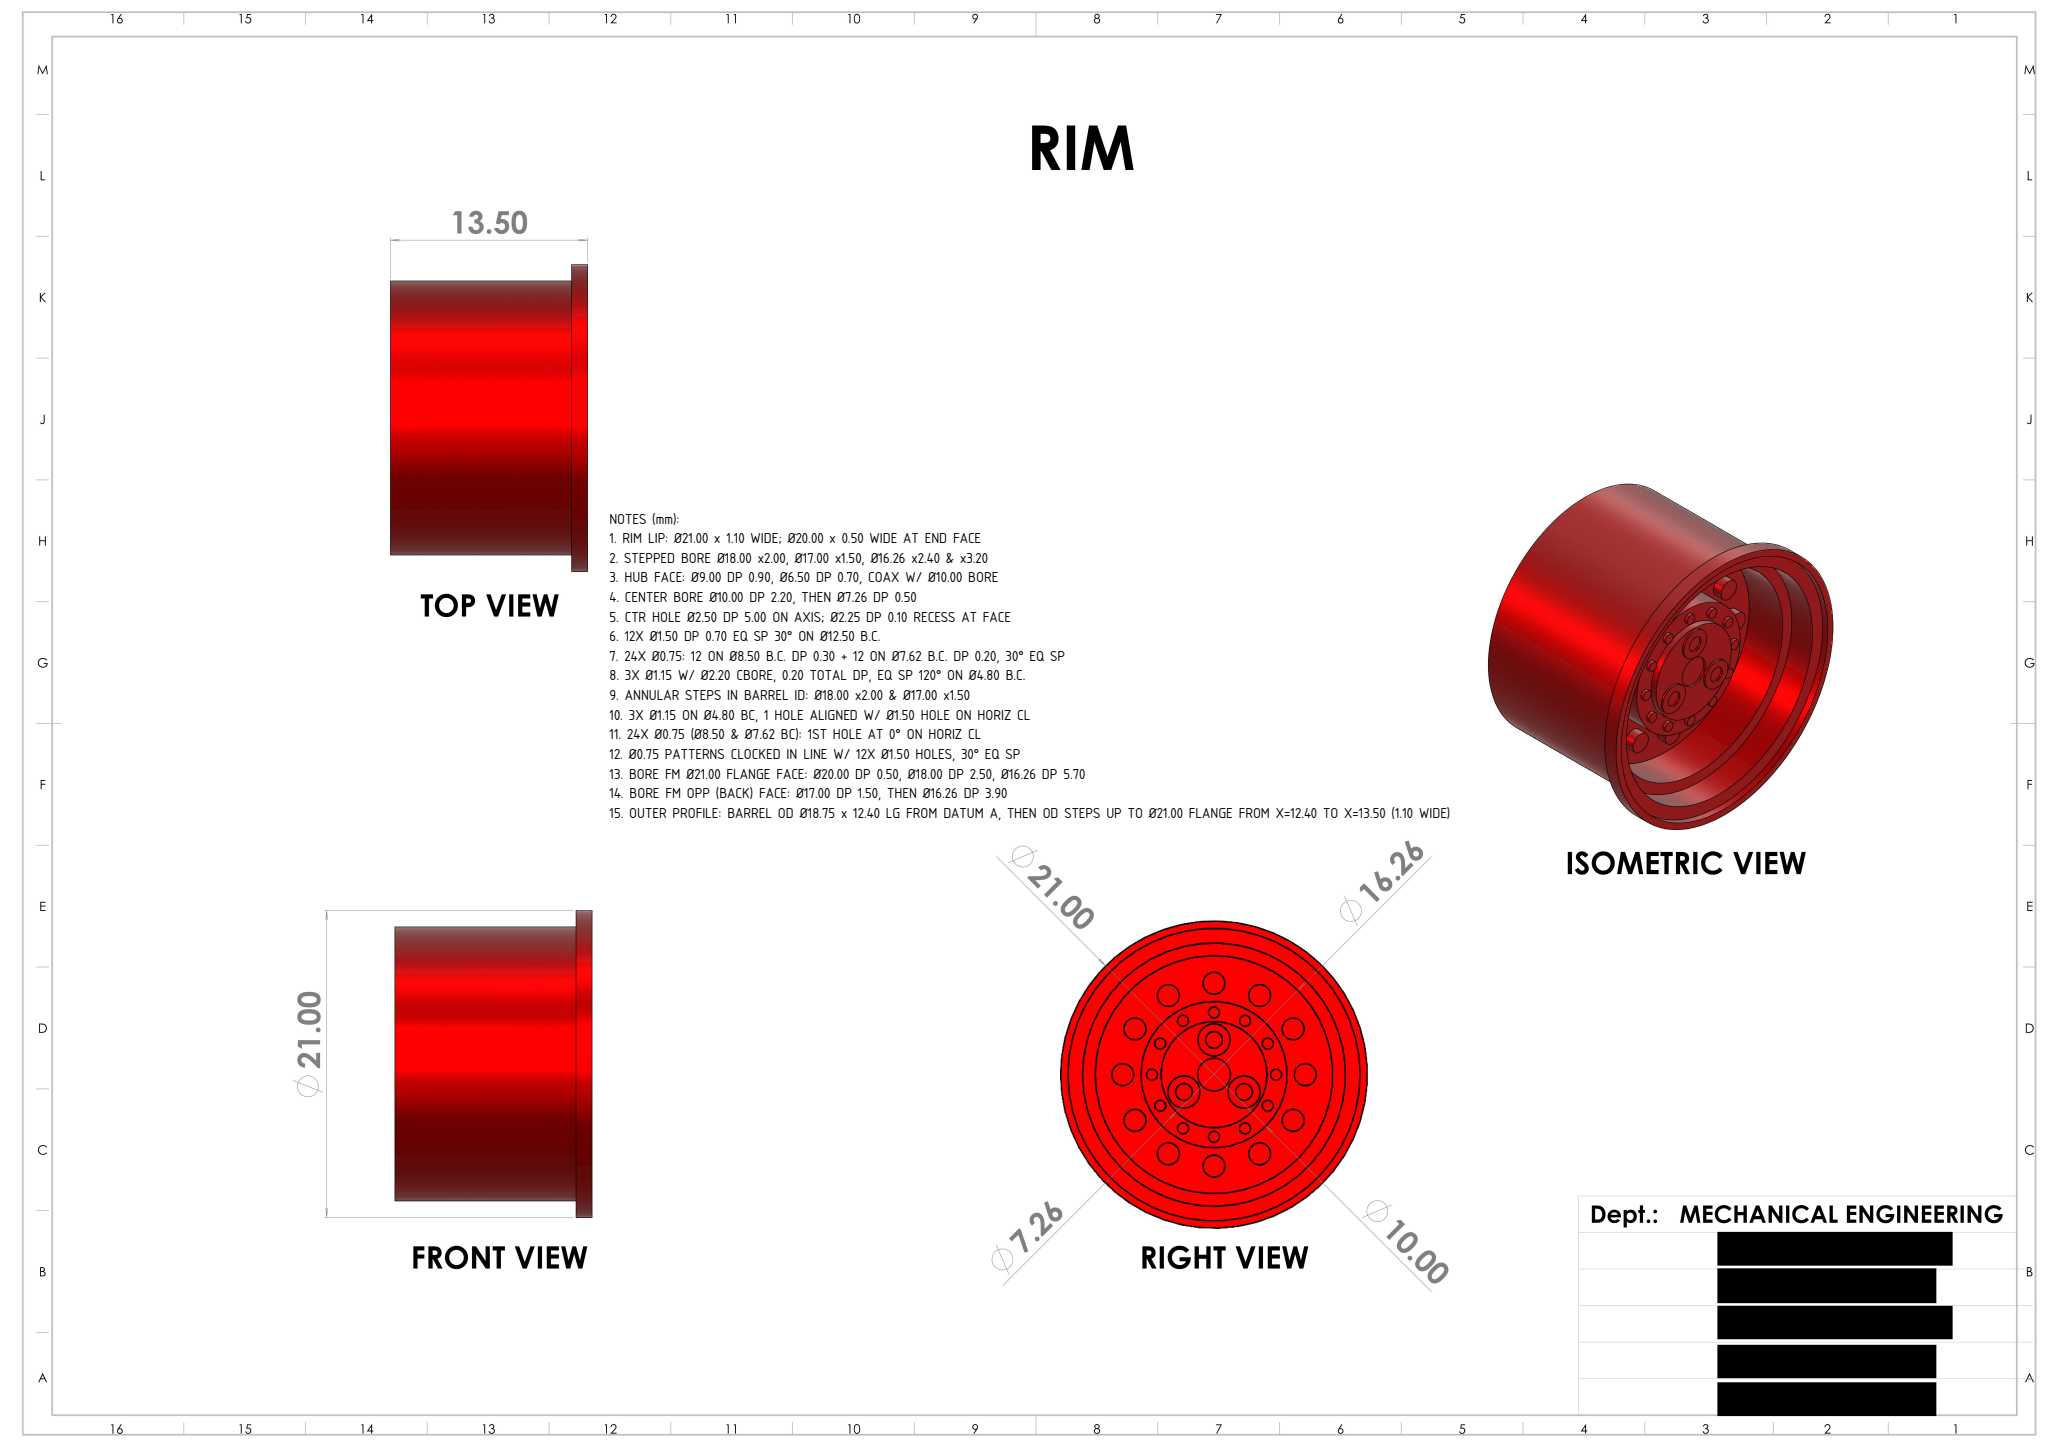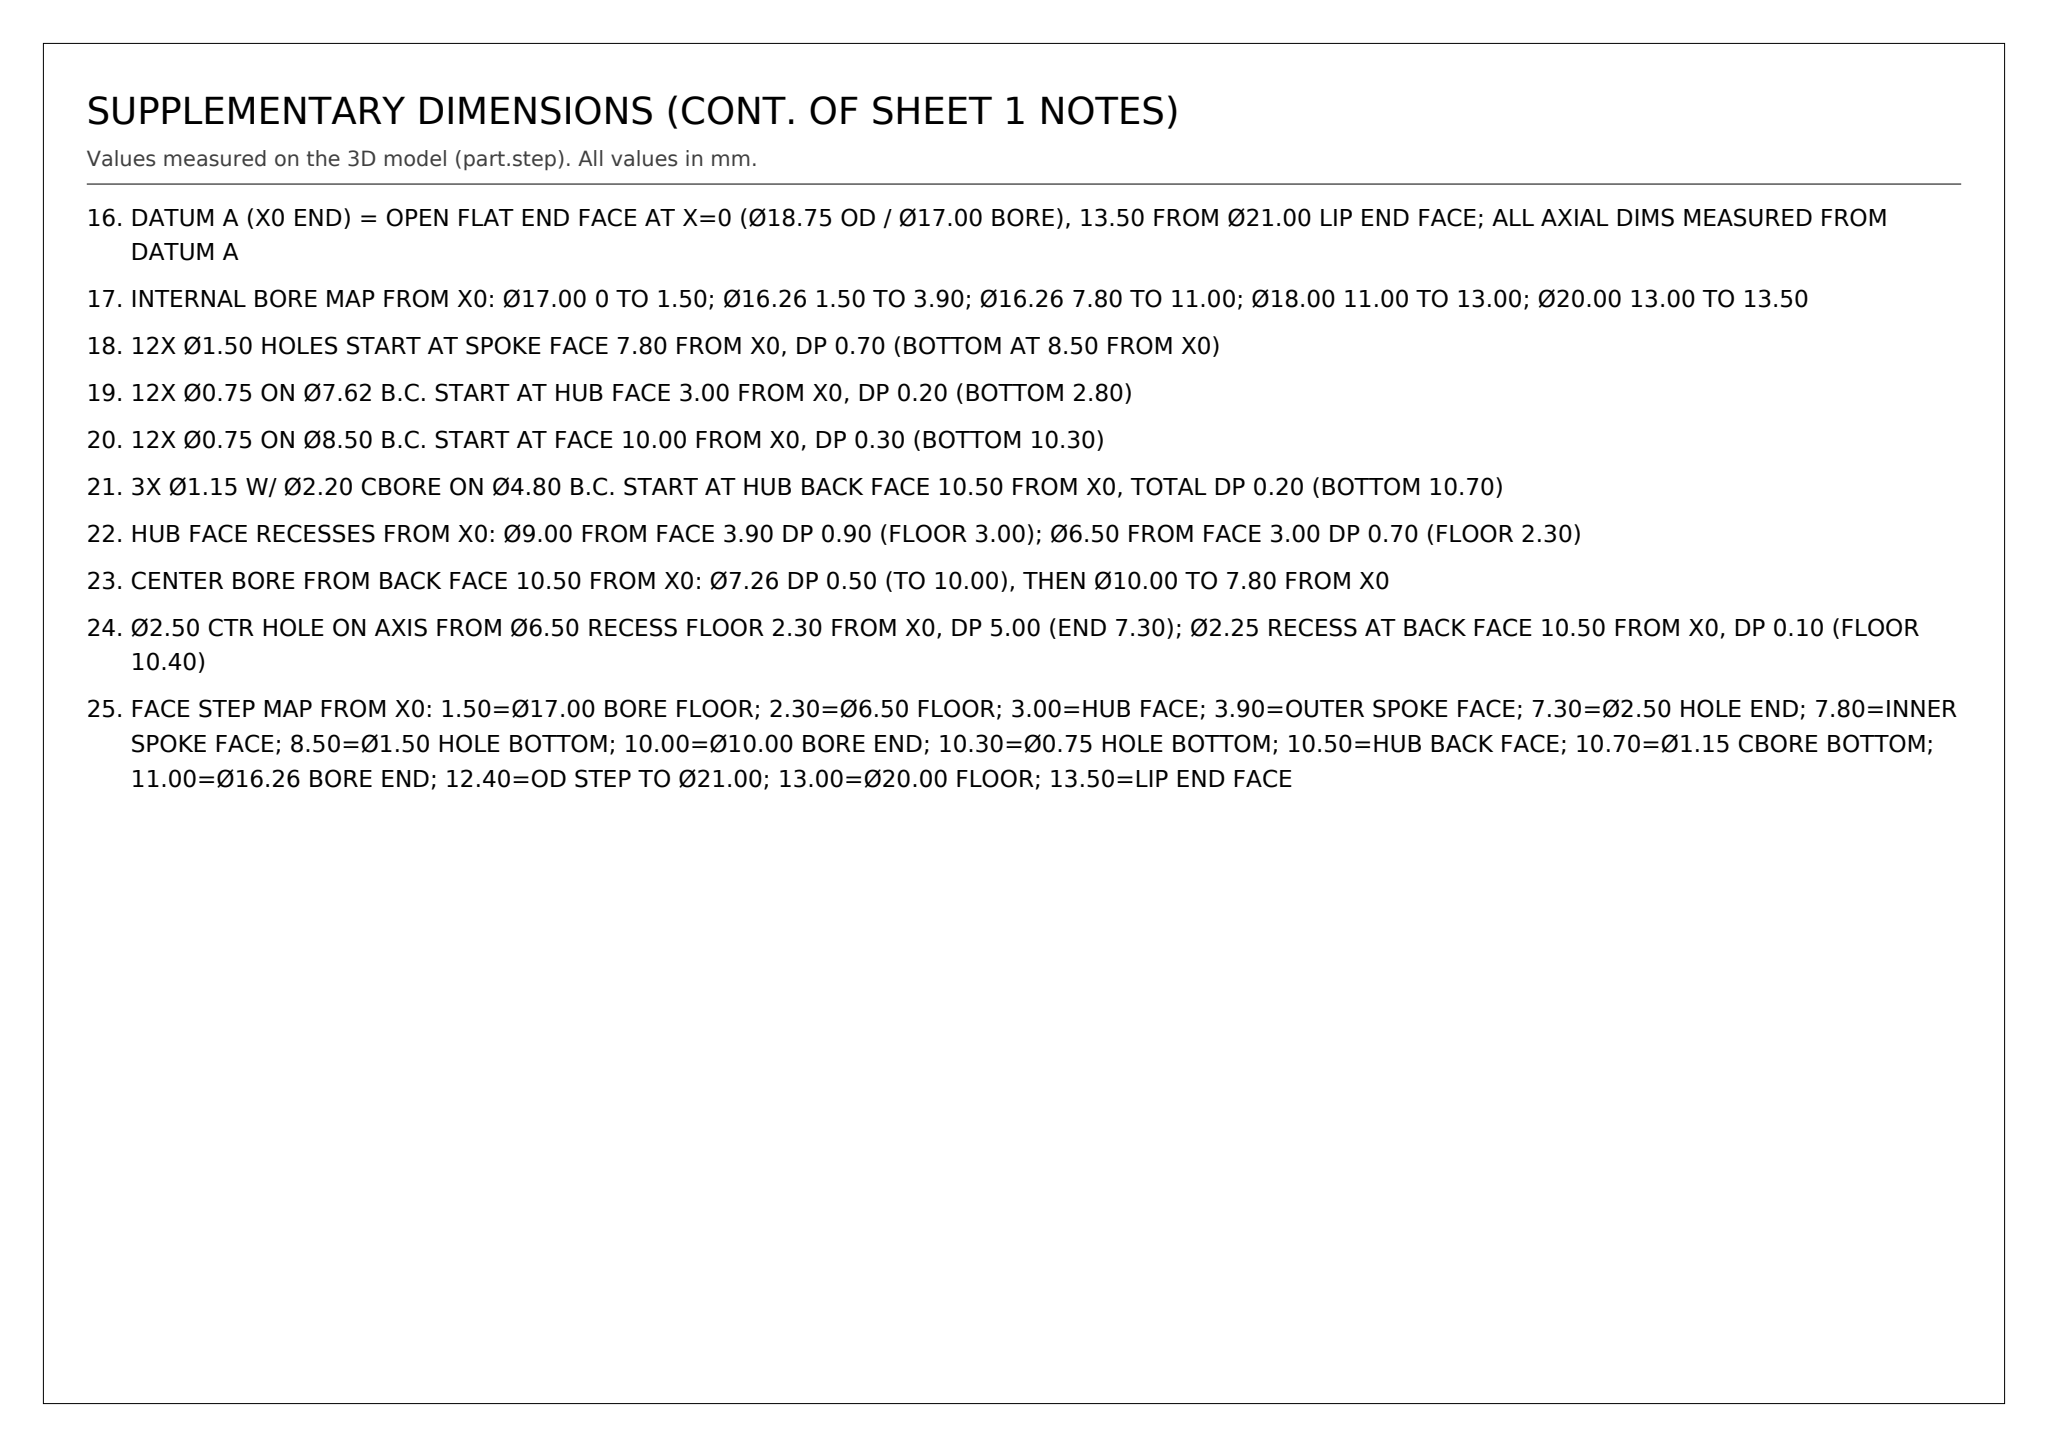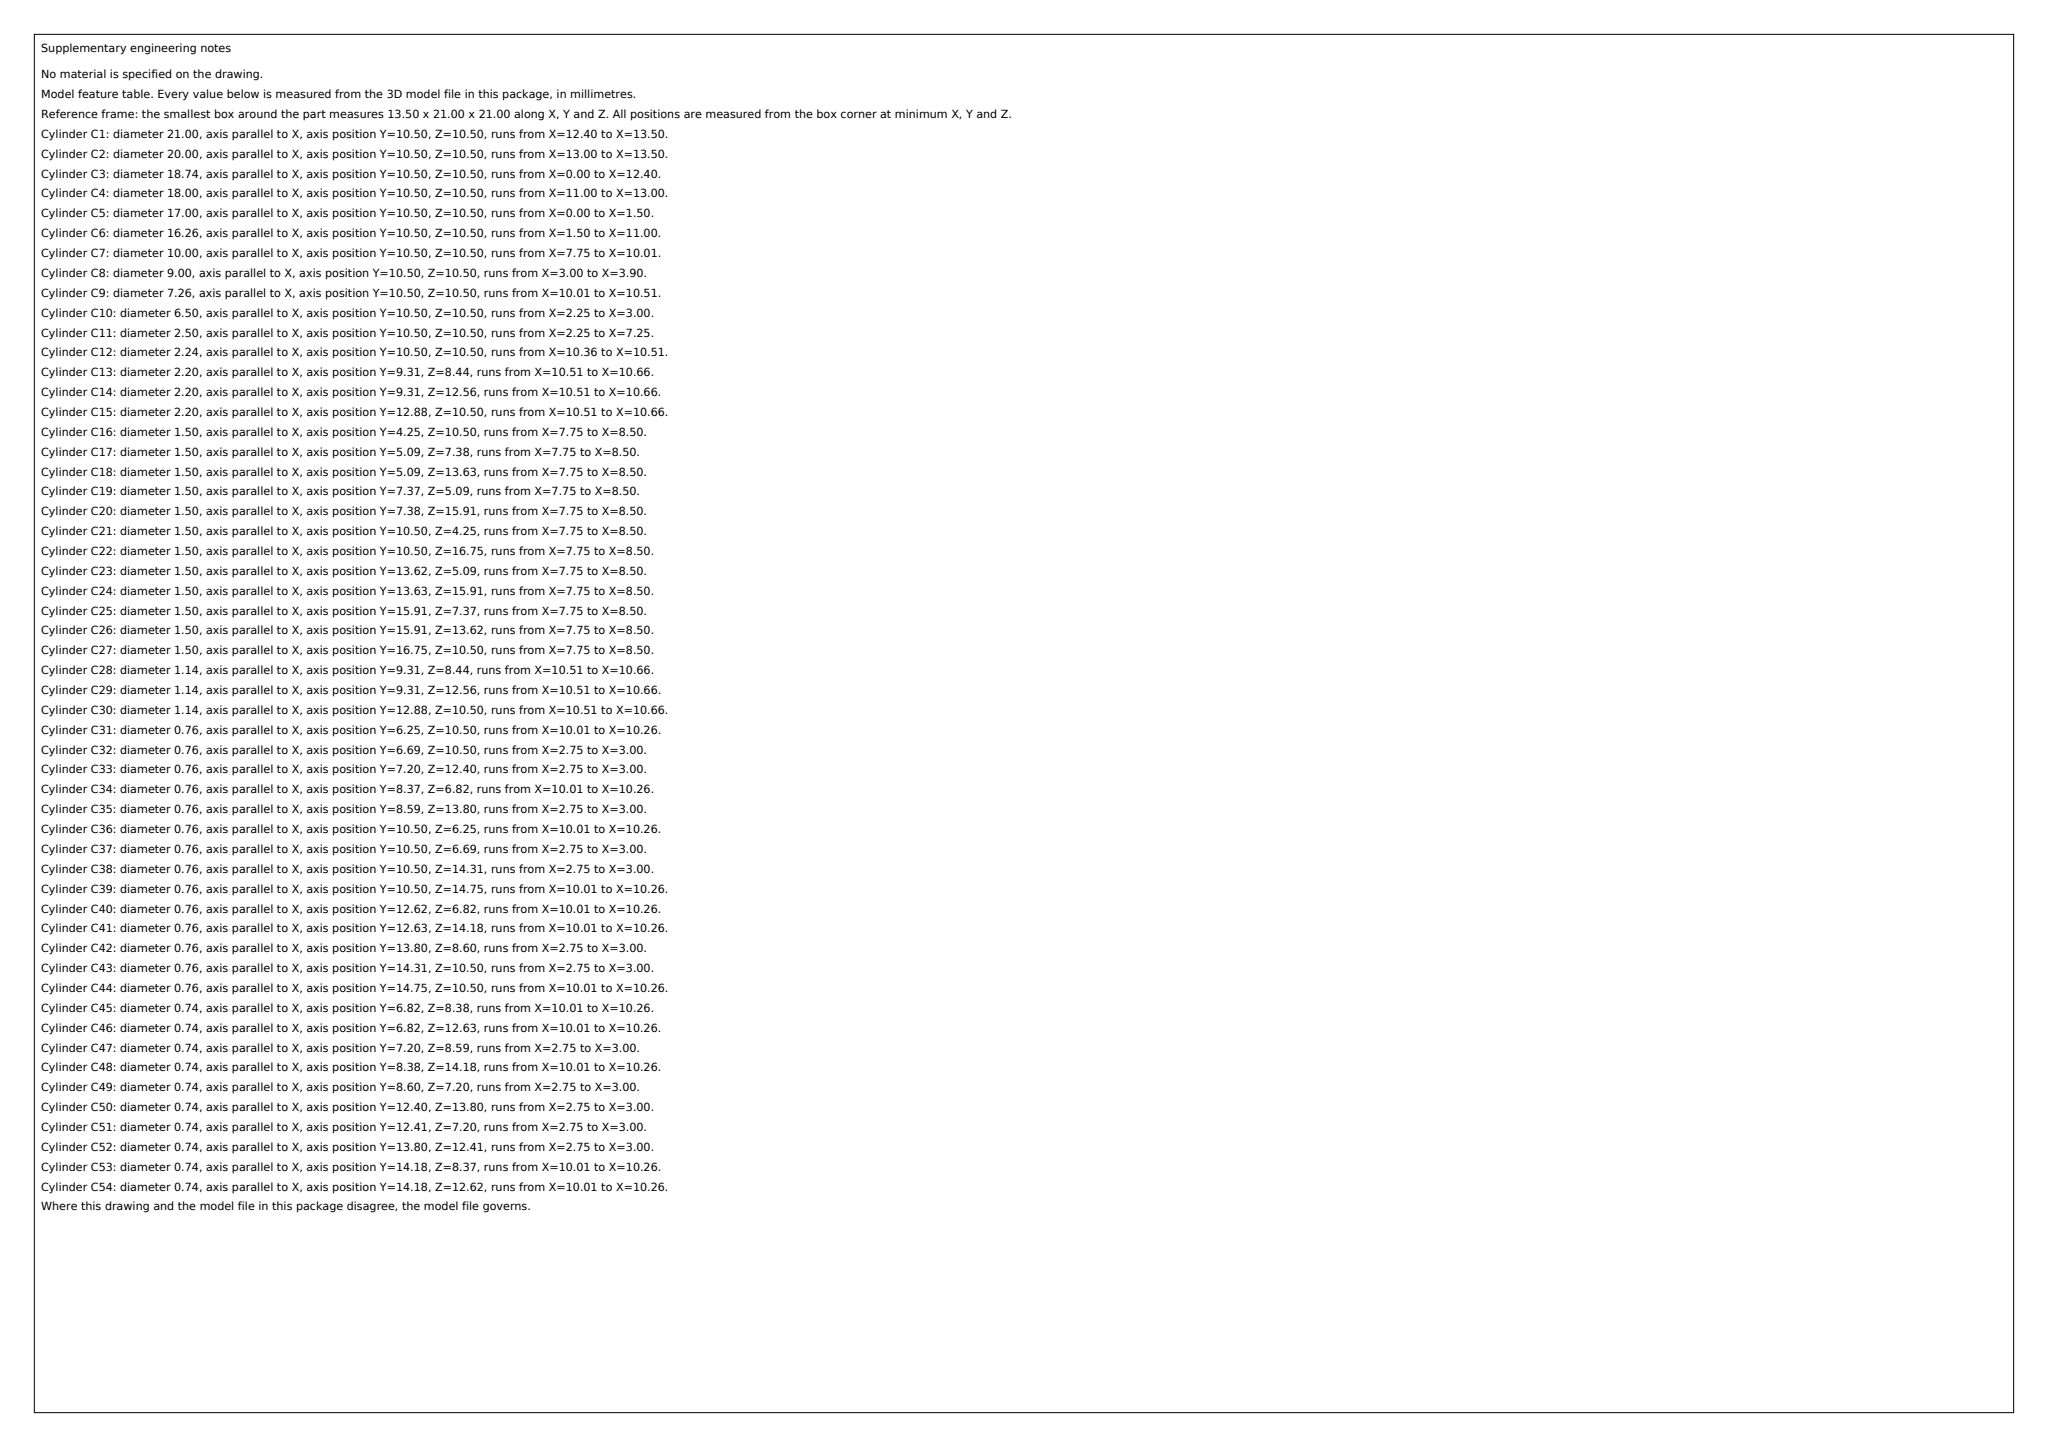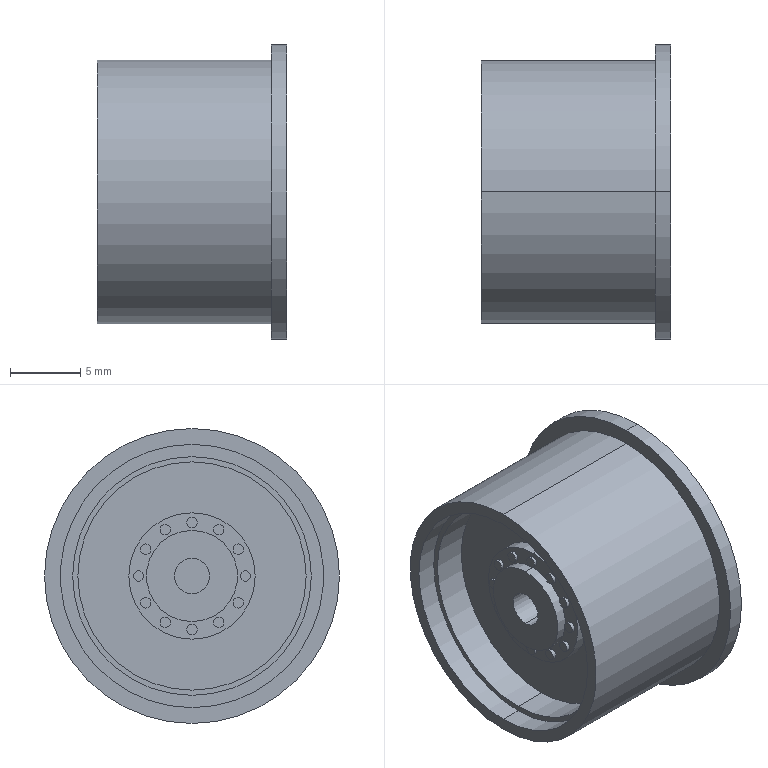Part | SolidWorks | mm | 1 solid | 166 faces | box 13.5 x 21 x 21 mm | volume 1900 mm3 | cylinder 110 | plane 56 | commonest cylinder face diameters 0.75 x48 1.5 x24 1.15 x6 2.2 x6 16.26 x4 2.5 x2 2.25 x2 21 x2
Drawing notes:
RIM LIP: Ø21.00 x 1.10 WIDE; Ø20.00 x 0.50 WIDE AT END FACE | from the solid: cyl [21.0,len 1.10] & [20.0,len 0.50]; planes x=12.40, 13.00, 13.50
STEPPED BORE Ø18.00 x2.00, Ø17.00 x1.50, Ø16.26 x2.40 & x3.20 | from the solid: bores: Ø18.00 x 11.00-13.00 (2.00); Ø17.00 x 0-1.50 (1.50); Ø16.26 x 1.50-3.90 (2.40) and x 7.80-11.00 (3.20)
HUB FACE: Ø9.00 DP 0.90, Ø6.50 DP 0.70, COAX W/ Ø10.00 BORE | from the solid: Ø9.00 x 3.00-3.90 (0.90); Ø6.50 x 2.30-3.00 (0.70); Ø10.00 bore x 7.80-10.00, all on axis y10.5 z10.5
CENTER BORE Ø10.00 DP 2.20, THEN Ø7.26 DP 0.50 | from the solid: Ø10.00 x 7.80-10.00 (2.20); Ø7.26 x 10.00-10.50 (0.50)
CTR HOLE Ø2.50 DP 5.00 ON AXIS; Ø2.25 DP 0.10 RECESS AT FACE | from the solid: Ø2.50 bore x 2.30-7.30 (5.00); Ø2.25 bore x 10.40-10.50 (0.10)
12X Ø1.50 DP 0.70 EQ SP 30° ON Ø12.50 B.C. | from the solid: 12X Ø1.50 x 7.80-8.50 (0.70), centers at radius 6.25 from axis (e.g. y10.5 z16.8; y15.9 z13.6)
24X Ø0.75: 12 ON Ø8.50 B.C. DP 0.30 + 12 ON Ø7.62 B.C. DP 0.20, 30° EQ SP | from the solid: 12X Ø0.75 x 10.00-10.30 (0.30) at r=4.25; 12X Ø0.75 x 2.80-3.00 (0.20) at r=3.81
3X Ø1.15 W/ Ø2.20 CBORE, 0.20 TOTAL DP, EQ SP 120° ON Ø4.80 B.C. | from the solid: 3X Ø2.20 and Ø1.15 x 10.50-10.70 (0.20) at (y12.9 z10.5), (y9.3 z12.6), (y9.3 z8.4) = r 2.40
ANNULAR STEPS IN BARREL ID: Ø18.00 x2.00 & Ø17.00 x1.50 | from the solid: cyls [18.0,len 2.0],[17.0,len 1.5] coax with Ø18.75 bore
3X Ø1.15 ON Ø4.80 BC, 1 HOLE ALIGNED W/ Ø1.50 HOLE ON HORIZ CL | from the solid: Ø1.15 holes at r=2.40 from axis (y12.9 z10.5 etc.), one at z=10.5 in line with Ø1.50 hole at y16.8 z10.5
24X Ø0.75 (Ø8.50 & Ø7.62 BC): 1ST HOLE AT 0° ON HORIZ CL | from the solid: Ø0.75 holes at r=4.25 (Ø8.50 BC) and r=3.81 (Ø7.62 BC) about center y10.5 z10.5; both sets at 0,30,60...330° (e.g. 14.75,10.5 and 14.31,10.5 on +Y horiz CL)
Ø0.75 PATTERNS CLOCKED IN LINE W/ 12X Ø1.50 HOLES, 30° EQ SP | from the solid: Ø1.50 holes r=6.25 at (16.75,10.5)=0°,(15.91,13.63)=30°...; same 0° start as both Ø0.75 bolt circles
BORE FM Ø21.00 FLANGE FACE: Ø20.00 DP 0.50, Ø18.00 DP 2.50, Ø16.26 DP 5.70 | from the solid: from x=13.50: Ø20.00 to 13.00 (0.50); Ø18.00 to 11.00 (2.50); Ø16.26 to 7.80 (5.70)
BORE FM OPP (BACK) FACE: Ø17.00 DP 1.50, THEN Ø16.26 DP 3.90 | from the solid: planes x0/1.5 = Ø17.00 x1.50; x1.5/3.9 = Ø16.26 x2.40; back face = x0, Ø18.75 barrel runs x0-12.4
OUTER PROFILE: BARREL OD Ø18.75 x 12.40 LG FROM DATUM A, THEN OD STEPS UP TO Ø21.00 FLANGE FROM X=12.40 TO X=13.50 (1.10 WIDE) | from the solid: cylinders Ø18.75 axis x L12.40 and Ø21.00 axis x L1.10; axis_plane x=12.4
DATUM A (X0 END) = OPEN FLAT END FACE AT X=0 (Ø18.75 OD / Ø17.00 BORE), 13.50 FROM Ø21.00 LIP END FACE; ALL AXIAL DIMS MEASURED FROM DATUM A | from the solid: axis_planes x=0.0 (extent y,z 1.1-19.9) and x=13.5; bbox_xyz x=13.50
INTERNAL BORE MAP FROM X0: Ø17.00 0 TO 1.50; Ø16.26 1.50 TO 3.90; Ø16.26 7.80 TO 11.00; Ø18.00 11.00 TO 13.00; Ø20.00 13.00 TO 13.50 | from the solid: hole/bore Ø17.0 x 0.0-1.5; Ø16.26 x 1.5-3.9; Ø16.26 x 7.8-11.0; Ø18.0 x 11.0-13.0; Ø20.0 x 13.0-13.5
12X Ø1.50 HOLES START AT SPOKE FACE 7.80 FROM X0, DP 0.70 (BOTTOM AT 8.50 FROM X0) | from the solid: cylinders Ø1.5 axis x from 7.8 to 8.5 (12 instances); axis_planes x=7.8 and x=8.5 pockets
12X Ø0.75 ON Ø7.62 B.C. START AT HUB FACE 3.00 FROM X0, DP 0.20 (BOTTOM 2.80) | from the solid: cylinders Ø0.75 axis x from 2.8 to 3.0 (12 instances, radius 3.8 from axis y10.5 z10.5); axis_plane x=3.0
12X Ø0.75 ON Ø8.50 B.C. START AT FACE 10.00 FROM X0, DP 0.30 (BOTTOM 10.30) | from the solid: cylinders Ø0.75 axis x from 10.0 to 10.3 (12 instances, radius ~4.3 from axis y10.5 z10.5); axis_plane x=10.0
3X Ø1.15 W/ Ø2.20 CBORE ON Ø4.80 B.C. START AT HUB BACK FACE 10.50 FROM X0, TOTAL DP 0.20 (BOTTOM 10.70) | from the solid: hole/bore Ø1.15 and Ø2.2 axis x from 10.5 to 10.7 at (y12.9,z10.5),(y9.3,z12.6),(y9.3,z8.4); axis_plane x=10.5
HUB FACE RECESSES FROM X0: Ø9.00 FROM FACE 3.90 DP 0.90 (FLOOR 3.00); Ø6.50 FROM FACE 3.00 DP 0.70 (FLOOR 2.30) | from the solid: cylinders Ø9.0 axis x 3.0-3.9; Ø6.5 axis x 2.3-3.0; axis_planes x=3.9, x=3.0, x=2.3
CENTER BORE FROM BACK FACE 10.50 FROM X0: Ø7.26 DP 0.50 (TO 10.00), THEN Ø10.00 TO 7.80 FROM X0 | from the solid: cylinders Ø7.26 axis x 10.0-10.5; Ø10.0 axis x 7.8-10.0; axis_planes x=10.5, x=10.0, x=7.8
Ø2.50 CTR HOLE ON AXIS FROM Ø6.50 RECESS FLOOR 2.30 FROM X0, DP 5.00 (END 7.30); Ø2.25 RECESS AT BACK FACE 10.50 FROM X0, DP 0.10 (FLOOR 10.40) | from the solid: hole/bore Ø2.5 axis x 2.3-7.3; hole/bore Ø2.25 axis x 10.4-10.5; axis_planes x=2.3, x=7.3, x=10.4, x=10.5
FACE STEP MAP FROM X0: 1.50=Ø17.00 BORE FLOOR; 2.30=Ø6.50 FLOOR; 3.00=HUB FACE; 3.90=OUTER SPOKE FACE; 7.30=Ø2.50 HOLE END; 7.80=INNER SPOKE FACE; 8.50=Ø1.50 HOLE BOTTOM; 10.00=Ø10.00 BORE END; 10.30=Ø0.75 HOLE BOTTOM; 10.50=HUB BACK FACE; 10.70=Ø1.15 CBORE BOTTOM; 11.00=Ø16.26 BORE END; 12.40=OD STEP TO Ø21.00; 13.00=Ø20.00 FLOOR; 13.50=LIP END FACE | from the solid: axis_planes normal x at offsets 1.5, 2.3, 3.0, 3.9, 7.3, 7.8, 8.5, 10.0, 10.3, 10.5, 10.7, 11.0, 12.4, 13.0, 13.5
build123d program:
from build123d import *

# Parameters (mm, degrees)
SKETCH2_R           = 0.75
BOSS_EXTRUDE1_DEPTH = 0.75
SKETCH3_R           = 0.375
BOSS_EXTRUDE2_DEPTH = 0.25
SKETCH4_R           = 1.125
CUT_EXTRUDE1_DEPTH  = 0.15
SKETCH5_R           = 1.1
SKETCH5_R_2         = 0.575
BOSS_EXTRUDE3_DEPTH = 0.15
SKETCH6_R           = 0.375
BOSS_EXTRUDE4_DEPTH = 0.25
SKETCH7_R           = 1.25
CUT_EXTRUDE2_DEPTH  = 5


with BuildPart() as part:
    # Sketch1 → Revolve1 (revolve)
    with BuildSketch(Plane.XY, mode=Mode.PRIVATE) as revolve1_sk:
        Polygon((0, 9.375), (-6.81, 9.375), (-6.81, 8.5), (-5.31, 8.5), (-5.31, 8.13), (-2.91, 8.13), (-2.91, 4.5), (-3.81, 4.5), (-3.81, 3.25), (-4.56, 3.25), (-4.56, 0), (3.7, 0), (3.7, 3.63), (3.2, 3.63), (3.2, 5), (0.94, 5), (0.94, 8.13), (4.19, 8.13), (4.19, 9), (6.19, 9), (6.19, 10), (6.69, 10), (6.69, 10.5), (5.59, 10.5), (5.59, 9.375), align=None)
    revolve(revolve1_sk.sketch.rotate(Axis((-4.56, 0, 0), (1, 0, 0)), 90), axis=Axis((-4.56, 0, 0), (1, 0, 0)))

    # Sketch2 → Boss-Extrude1 (add)
    with BuildSketch(Plane(origin=(0.94, 0, 0), x_dir=(0, 0, -1), z_dir=(1, 0, 0))):
        with Locations(Location((0, 6.25, 0), (0, 0, 180))):
            Circle(SKETCH2_R)
        with Locations(Location((3.125, 5.413, 0), (0, 0, 180))):
            Circle(SKETCH2_R)
        with Locations(Location((5.413, 3.125, 0), (0, 0, 180))):
            Circle(SKETCH2_R)
        with Locations(Location((6.25, 0, 0), (0, 0, 180))):
            Circle(SKETCH2_R)
        with Locations(Location((5.413, -3.125, 0), (0, 0, 180))):
            Circle(SKETCH2_R)
        with Locations(Location((3.125, -5.413, 0), (0, 0, 180))):
            Circle(SKETCH2_R)
        with Locations(Location((0, -6.25, 0), (0, 0, 180))):
            Circle(SKETCH2_R)
        with Locations(Location((-3.125, -5.413, 0), (0, 0, 180))):
            Circle(SKETCH2_R)
        with Locations(Location((-5.413, -3.125, 0), (0, 0, 180))):
            Circle(SKETCH2_R)
        with Locations(Location((-6.25, 0, 0), (0, 0, 180))):
            Circle(SKETCH2_R)
        with Locations(Location((-5.413, 3.125, 0), (0, 0, 180))):
            Circle(SKETCH2_R)
        with Locations(Location((-3.125, 5.413, 0), (0, 0, 180))):
            Circle(SKETCH2_R)
    extrude(amount=BOSS_EXTRUDE1_DEPTH)

    # Sketch3 → Boss-Extrude2 (add)
    with BuildSketch(Plane(origin=(3.2, 0, 0), x_dir=(0, 0, -1), z_dir=(1, 0, 0))):
        with Locations(Location((0, 4.25, 0), (0, 0, 180))):
            Circle(SKETCH3_R)
        with Locations(Location((2.125, 3.681, 0), (0, 0, 180))):
            Circle(SKETCH3_R)
        with Locations(Location((3.681, 2.125, 0), (0, 0, 180))):
            Circle(SKETCH3_R)
        with Locations(Location((4.25, 0, 0), (0, 0, 180))):
            Circle(SKETCH3_R)
        with Locations(Location((3.681, -2.125, 0), (0, 0, 180))):
            Circle(SKETCH3_R)
        with Locations(Location((2.125, -3.681, 0), (0, 0, 180))):
            Circle(SKETCH3_R)
        with Locations(Location((0, -4.25, 0), (0, 0, 180))):
            Circle(SKETCH3_R)
        with Locations(Location((-2.125, -3.681, 0), (0, 0, 180))):
            Circle(SKETCH3_R)
        with Locations(Location((-3.681, -2.125, 0), (0, 0, 180))):
            Circle(SKETCH3_R)
        with Locations(Location((-4.25, 0, 0), (0, 0, 180))):
            Circle(SKETCH3_R)
        with Locations(Location((-3.681, 2.125, 0), (0, 0, 180))):
            Circle(SKETCH3_R)
        with Locations(Location((-2.125, 3.681, 0), (0, 0, 180))):
            Circle(SKETCH3_R)
    extrude(amount=BOSS_EXTRUDE2_DEPTH)

    # Sketch4 → Cut-Extrude1 (cut)
    with BuildSketch(Plane(origin=(3.7, 0, 0), x_dir=(0, 0, -1), z_dir=(1, 0, 0))):
        Circle(SKETCH4_R)
    extrude(amount=-CUT_EXTRUDE1_DEPTH, mode=Mode.SUBTRACT)

    # Sketch5 → Boss-Extrude3 (add)
    # profile 1 of 3: a face of its own
    with BuildSketch(Plane(origin=(3.7, 0, 0), x_dir=(0, 0, -1), z_dir=(1, 0, 0))):
        with Locations(Location((0, 2.375, 0), (0, 0, 180))):
            Circle(SKETCH5_R)
        with Locations((0, 2.375)):
            Circle(SKETCH5_R_2, mode=Mode.SUBTRACT)
    # profile 2 of 3: a face of its own
    with BuildSketch(Plane(origin=(3.7, 0, 0), x_dir=(0, 0, -1), z_dir=(1, 0, 0))):
        with Locations(Location((2.057, -1.188, 0), (0, 0, 180))):
            Circle(SKETCH5_R)
        with Locations((2.057, -1.188)):
            Circle(SKETCH5_R_2, mode=Mode.SUBTRACT)
    # profile 3 of 3: a face of its own
    with BuildSketch(Plane(origin=(3.7, 0, 0), x_dir=(0, 0, -1), z_dir=(1, 0, 0))):
        with Locations(Location((-2.057, -1.188, 0), (0, 0, 180))):
            Circle(SKETCH5_R)
        with Locations((-2.057, -1.188)):
            Circle(SKETCH5_R_2, mode=Mode.SUBTRACT)
    extrude(amount=BOSS_EXTRUDE3_DEPTH)

    # Sketch6 → Boss-Extrude4 (add)
    with BuildSketch(Plane.ZY.offset(3.81)):
        with Locations(Location((0, 3.81, 0), (0, 0, 180))):
            Circle(SKETCH6_R)
        with Locations(Location((1.905, 3.3, 0), (0, 0, 180))):
            Circle(SKETCH6_R)
        with Locations(Location((3.3, 1.905, 0), (0, 0, 180))):
            Circle(SKETCH6_R)
        with Locations(Location((3.81, 0, 0), (0, 0, 180))):
            Circle(SKETCH6_R)
        with Locations(Location((3.3, -1.905, 0), (0, 0, 180))):
            Circle(SKETCH6_R)
        with Locations(Location((1.905, -3.3, 0), (0, 0, 180))):
            Circle(SKETCH6_R)
        with Locations(Location((0, -3.81, 0), (0, 0, 180))):
            Circle(SKETCH6_R)
        with Locations(Location((-1.905, -3.3, 0), (0, 0, 180))):
            Circle(SKETCH6_R)
        with Locations(Location((-3.3, -1.905, 0), (0, 0, 180))):
            Circle(SKETCH6_R)
        with Locations(Location((-3.81, 0, 0), (0, 0, 180))):
            Circle(SKETCH6_R)
        with Locations(Location((-3.3, 1.905, 0), (0, 0, 180))):
            Circle(SKETCH6_R)
        with Locations(Location((-1.905, 3.3, 0), (0, 0, 180))):
            Circle(SKETCH6_R)
    extrude(amount=BOSS_EXTRUDE4_DEPTH)

    # Sketch7 → Cut-Extrude2 (cut)
    with BuildSketch(Plane.ZY.offset(4.56)):
        Circle(SKETCH7_R)
    extrude(amount=-CUT_EXTRUDE2_DEPTH, mode=Mode.SUBTRACT)


solid = part.part